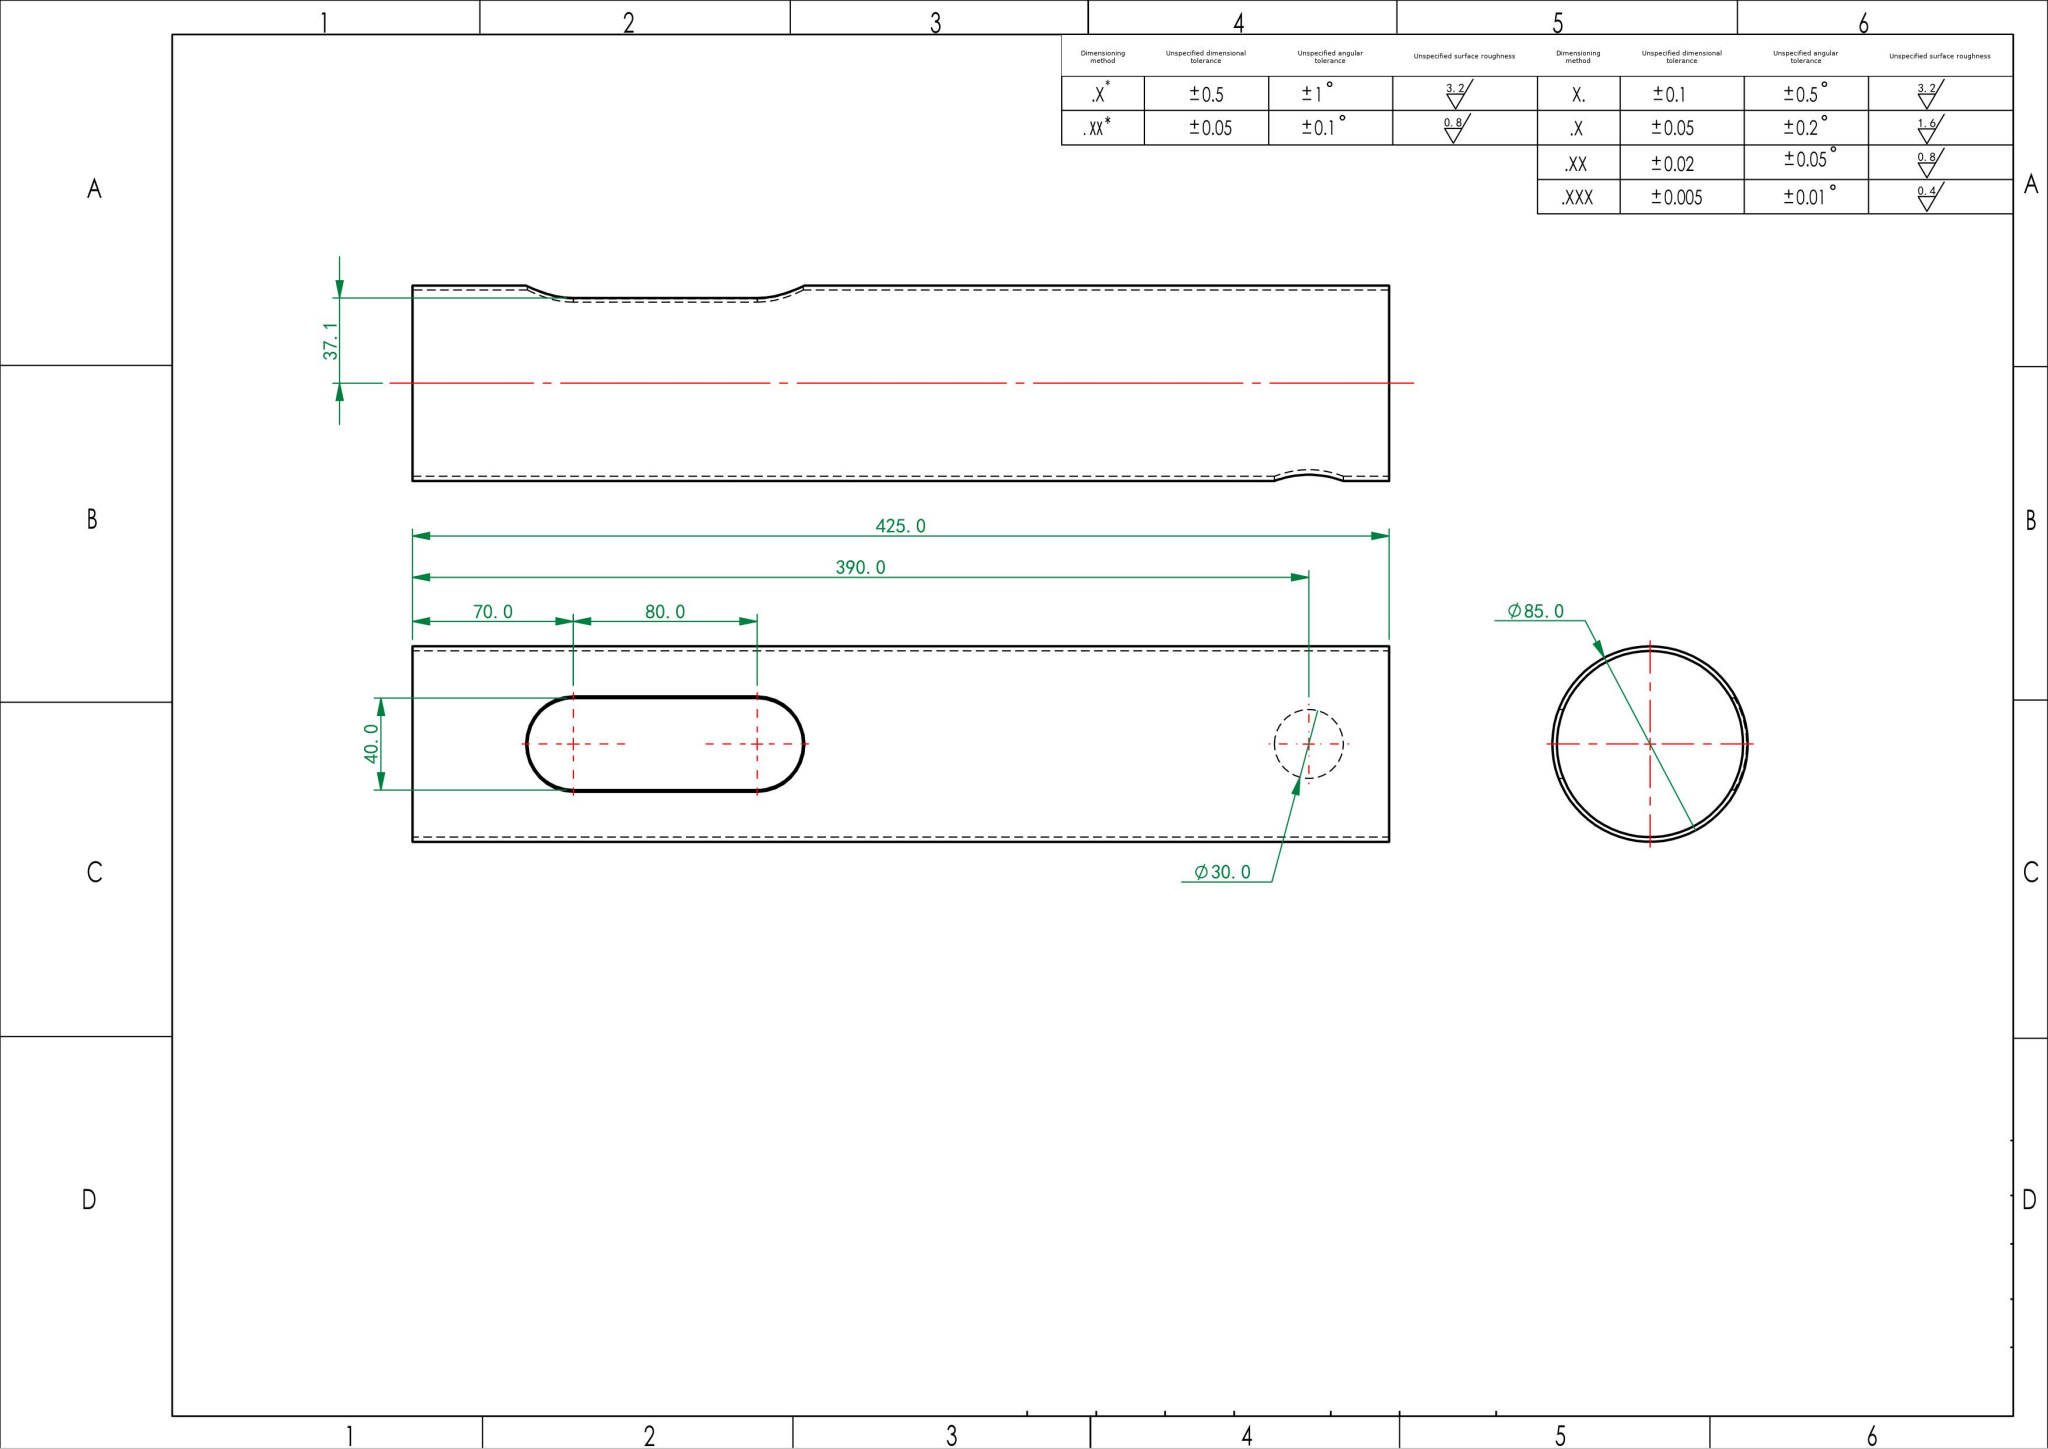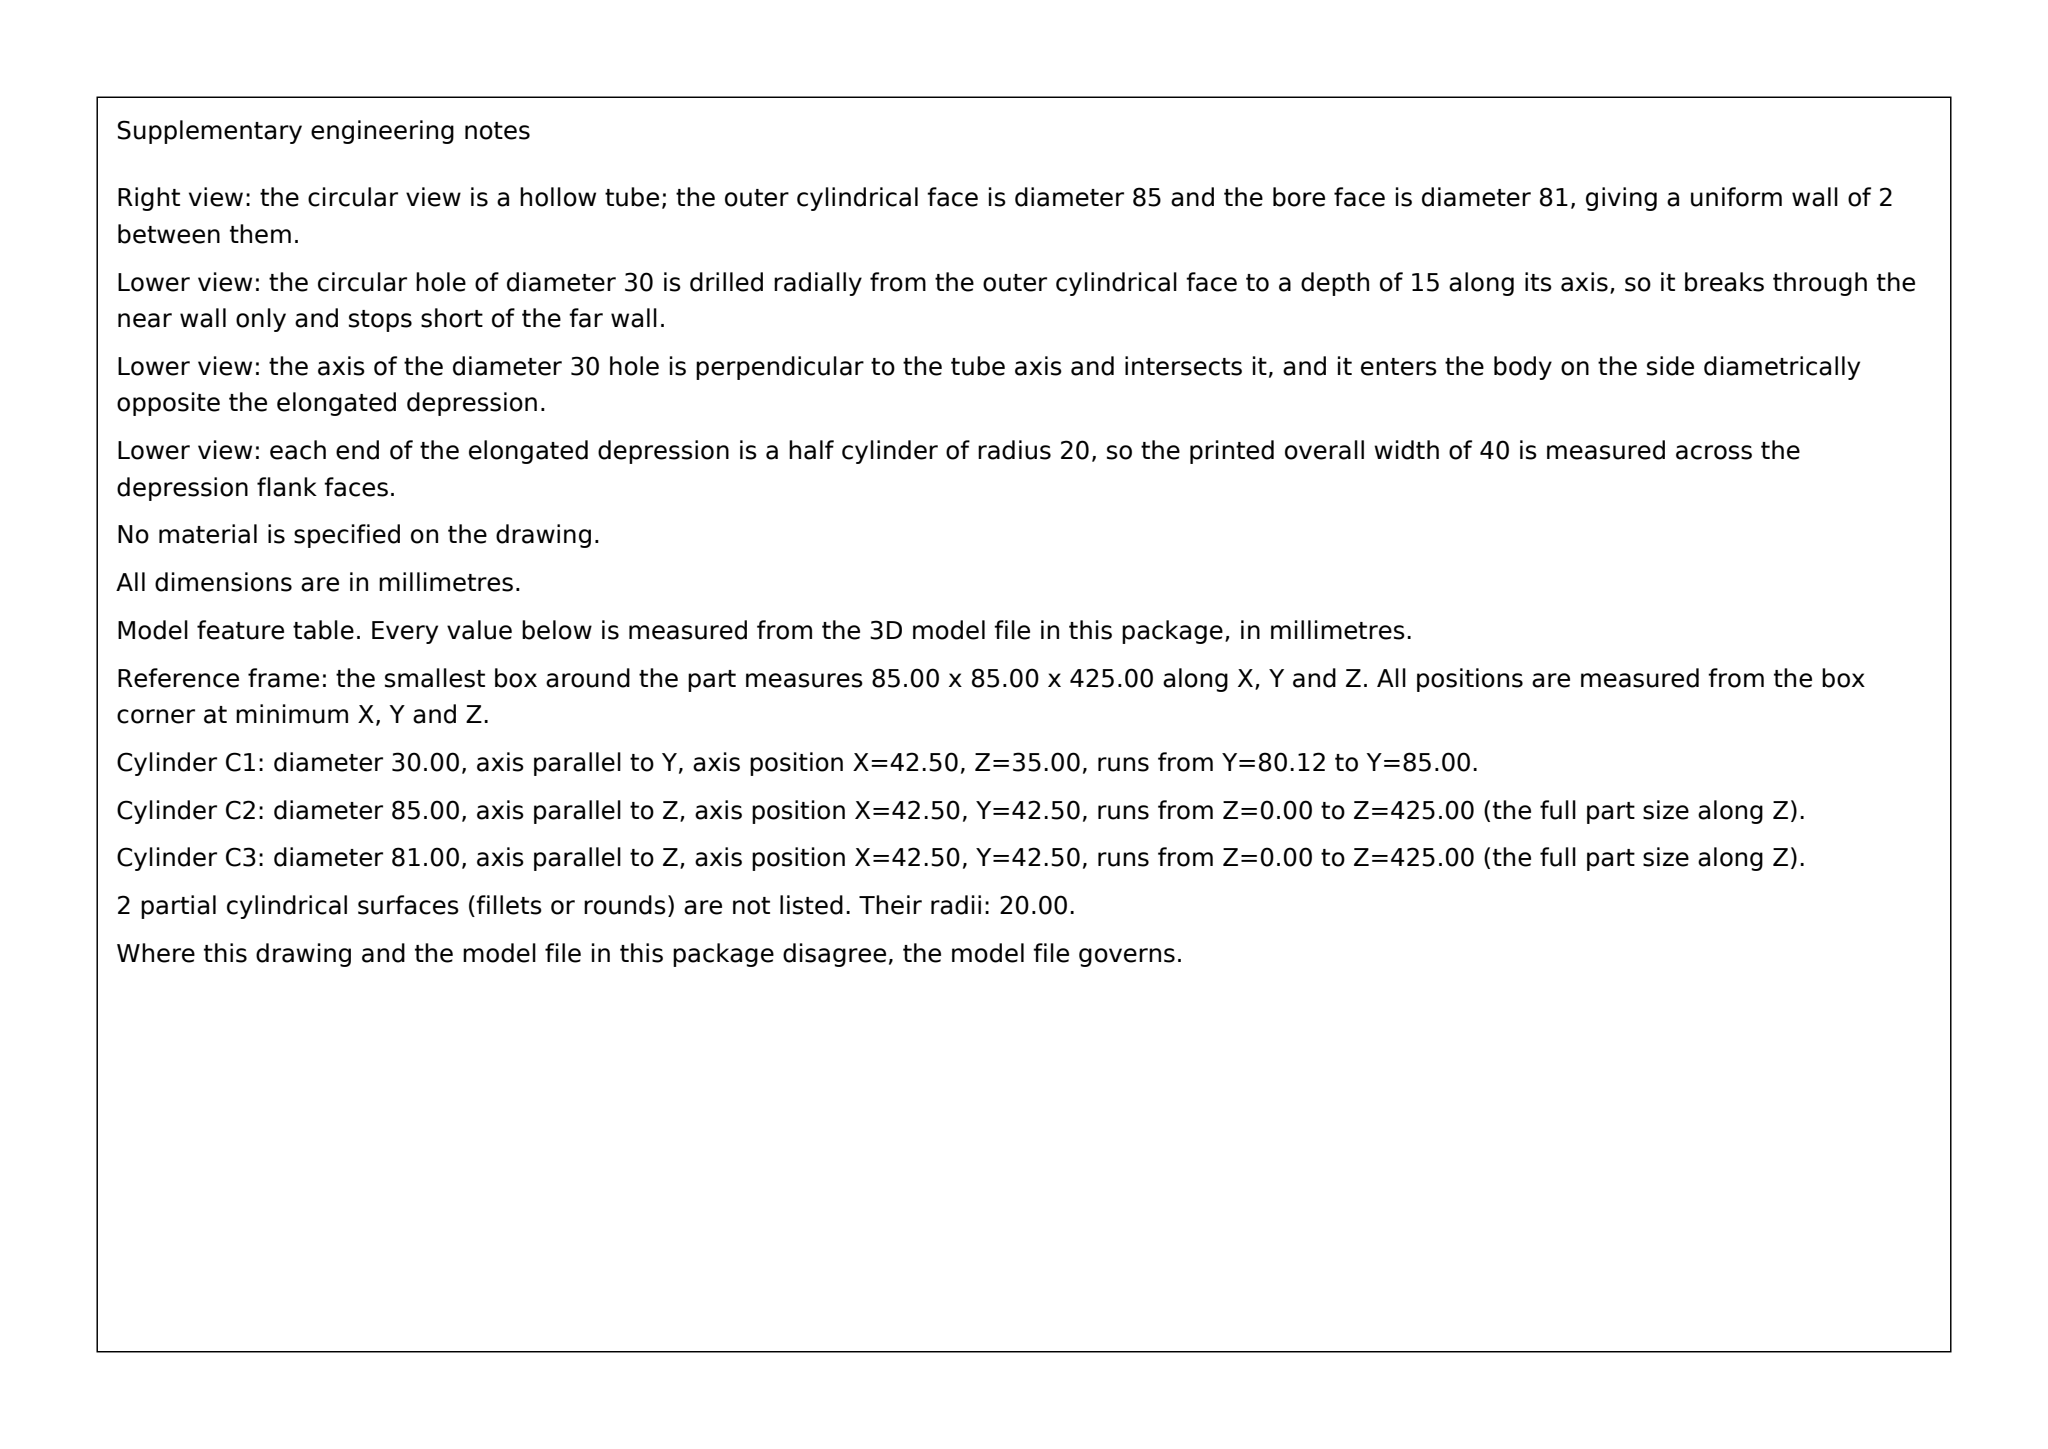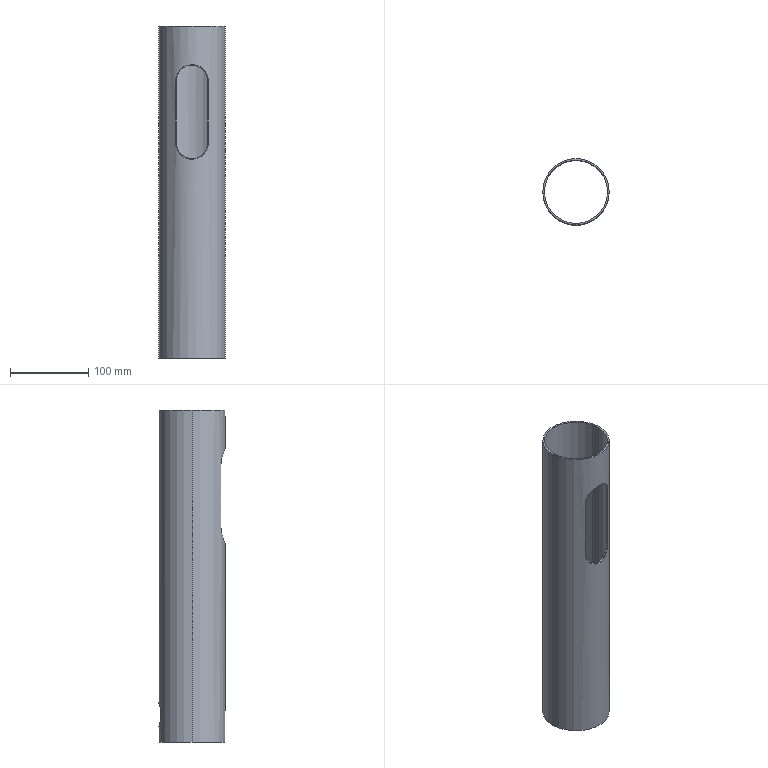Part | SolidWorks | mm | 1 solid | 17 faces | box 85 x 85 x 425 mm | volume 210854 mm3 | cylinder 9 | plane 6 | spline 2 | commonest cylinder face diameters 40 x3 30 x2 81 x2 85 x2
Drawing notes:
SECTION VIEW: BORE Ø81.0 THRU, 425.0 LG (WALL 2.0) | from the solid: cylinder dia 81.0 axis z, pos [42.5,42.5], length 425.0; OD 85.0 same axis